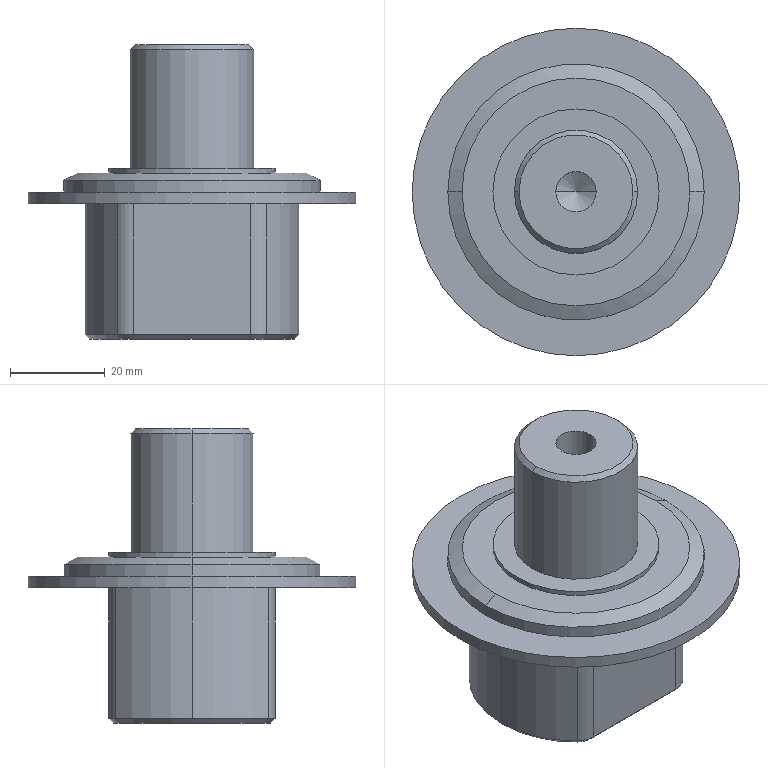Component | SolidWorks | 12AFlatGrooveSmallWheel-MillingAxis-1_12ASmallStraighteningWheelAxis-1 | 1 solid | 52 faces | volume 66562 mm3 | cylinder 23 | cone 19 | plane 10 | commonest cylinder face diameters 8.5 x8 10 x4 45 x3 69 x2 54 x2 35 x2 26 x2 | material 45